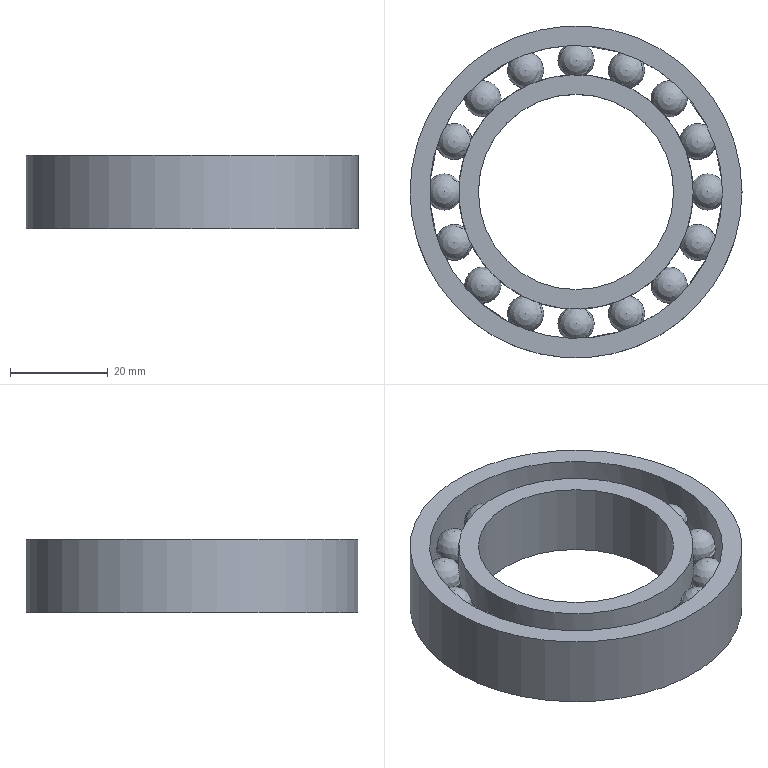Component | NX | GUNDONGZHOUCHENG | 1 solid | 41 faces | volume 23648 mm3 | sphere 16 | torus 16 | cylinder 5 | plane 4 | commonest cylinder face diameters 48 x2 40 x1 68 x1 60 x1